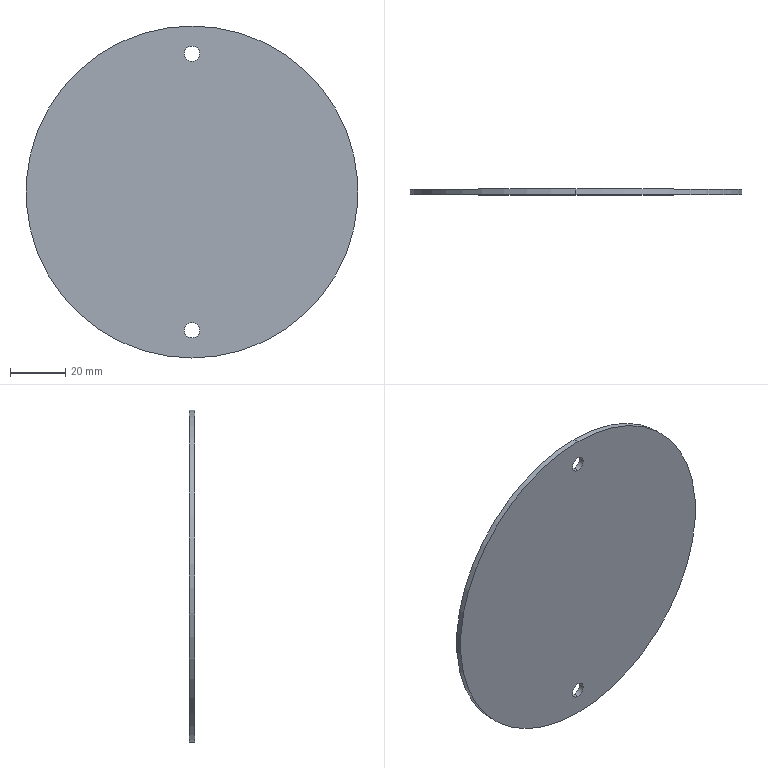Component | SolidWorks | YC1-25-01-08OilHoleCover-1 | 1 solid | 8 faces | box 120 x 2 x 120 mm | volume 22524 mm3 | cylinder 6 | plane 2 | commonest cylinder face diameters 5.5 x4 120 x2 | material Plain Carbon Steel
STEP:
#1=CARTESIAN_POINT('',(-19.291,153.78,-19.665));
#2=VERTEX_POINT('',#1);
#3=CARTESIAN_POINT('',(-19.291,153.78,-24.39));
#4=VERTEX_POINT('',#3);
#5=CARTESIAN_POINT('',(-19.291,153.78,-22.028));
#6=DIRECTION('',(0.,1.,0.));
#7=DIRECTION('',(0.,0.,-1.));
#8=AXIS2_PLACEMENT_3D('',#5,#6,#7);
#9=CIRCLE('',#8,2.362);
#10=EDGE_CURVE('',#2,#4,#9,.T.);
#11=ORIENTED_EDGE('',*,*,#10,.F.);
#12=CARTESIAN_POINT('',(-19.291,153.701,-19.665));
#13=VERTEX_POINT('',#12);
#14=CARTESIAN_POINT('',(-19.291,153.78,-19.665));
#15=DIRECTION('',(0.,-1.,0.));
#16=VECTOR('',#15,39.37);
#17=LINE('',#14,#16);
#18=EDGE_CURVE('',#2,#13,#17,.T.);
#19=ORIENTED_EDGE('',*,*,#18,.T.);
#20=CARTESIAN_POINT('',(-19.291,153.701,-24.39));
#21=VERTEX_POINT('',#20);
#22=CARTESIAN_POINT('',(-19.291,153.701,-22.028));
#23=DIRECTION('',(0.,1.,0.));
#24=DIRECTION('',(0.,0.,-1.));
#25=AXIS2_PLACEMENT_3D('',#22,#23,#24);
#26=CIRCLE('',#25,2.362);
#27=EDGE_CURVE('',#13,#21,#26,.T.);
#28=ORIENTED_EDGE('',*,*,#27,.T.);
#29=CARTESIAN_POINT('',(-19.291,153.78,-24.39));
#30=DIRECTION('',(0.,-1.,0.));
#31=VECTOR('',#30,39.37);
#32=LINE('',#29,#31);
#33=EDGE_CURVE('',#4,#21,#32,.T.);
#34=ORIENTED_EDGE('',*,*,#33,.F.);
#35=EDGE_LOOP('',(#11,#19,#28,#34));
#36=FACE_OUTER_BOUND('',#35,.T.);
#37=CARTESIAN_POINT('',(-19.291,153.78,-22.028));
#38=DIRECTION('',(0.,-1.,0.));
#39=DIRECTION('',(0.,0.,-1.));
#40=AXIS2_PLACEMENT_3D('',#37,#38,#39);
#41=CYLINDRICAL_SURFACE('',#40,2.362);
#42=ADVANCED_FACE('',(#36),#41,.T.);
#43=CARTESIAN_POINT('',(-19.291,153.701,-24.104));
#44=VERTEX_POINT('',#43);
#45=CARTESIAN_POINT('',(-19.291,153.701,-23.888));
#46=VERTEX_POINT('',#45);
#47=CARTESIAN_POINT('',(-19.291,153.701,-23.996));
#48=DIRECTION('',(0.,1.,0.));
#49=DIRECTION('',(0.,0.,1.));
#50=AXIS2_PLACEMENT_3D('',#47,#48,#49);
#51=CIRCLE('',#50,0.1083);
#52=EDGE_CURVE('',#44,#46,#51,.T.);
#53=ORIENTED_EDGE('',*,*,#52,.F.);
#54=CARTESIAN_POINT('',(-19.291,153.78,-24.104));
#55=VERTEX_POINT('',#54);
#56=CARTESIAN_POINT('',(-19.291,153.78,-24.104));
#57=DIRECTION('',(0.,1.,0.));
#58=VECTOR('',#57,39.37);
#59=LINE('',#56,#58);
#60=EDGE_CURVE('',#44,#55,#59,.T.);
#61=ORIENTED_EDGE('',*,*,#60,.T.);
#62=CARTESIAN_POINT('',(-19.291,153.78,-23.888));
#63=VERTEX_POINT('',#62);
#64=CARTESIAN_POINT('',(-19.291,153.78,-23.996));
#65=DIRECTION('',(0.,-1.,0.));
#66=DIRECTION('',(0.,0.,1.));
#67=AXIS2_PLACEMENT_3D('',#64,#65,#66);
#68=CIRCLE('',#67,0.1083);
#69=EDGE_CURVE('',#63,#55,#68,.T.);
#70=ORIENTED_EDGE('',*,*,#69,.F.);
#71=CARTESIAN_POINT('',(-19.291,153.78,-23.888));
#72=DIRECTION('',(0.,1.,0.));
#73=VECTOR('',#72,39.37);
#74=LINE('',#71,#73);
#75=EDGE_CURVE('',#46,#63,#74,.T.);
#76=ORIENTED_EDGE('',*,*,#75,.F.);
#77=EDGE_LOOP('',(#53,#61,#70,#76));
#78=FACE_OUTER_BOUND('',#77,.T.);
#79=CARTESIAN_POINT('',(-19.291,153.78,-23.996));
#80=DIRECTION('',(0.,1.,0.));
#81=DIRECTION('',(0.,0.,1.));
#82=AXIS2_PLACEMENT_3D('',#79,#80,#81);
#83=CYLINDRICAL_SURFACE('',#82,0.1083);
#84=ADVANCED_FACE('',(#78),#83,.F.);
#85=CARTESIAN_POINT('',(-19.291,153.701,-20.167));
#86=VERTEX_POINT('',#85);
#87=CARTESIAN_POINT('',(-19.291,153.701,-19.951));
#88=VERTEX_POINT('',#87);
#89=CARTESIAN_POINT('',(-19.291,153.701,-20.059));
#90=DIRECTION('',(0.,1.,0.));
#91=DIRECTION('',(0.,0.,1.));
#92=AXIS2_PLACEMENT_3D('',#89,#90,#91);
#93=CIRCLE('',#92,0.1083);
#94=EDGE_CURVE('',#86,#88,#93,.T.);
#95=ORIENTED_EDGE('',*,*,#94,.F.);
#96=CARTESIAN_POINT('',(-19.291,153.78,-20.167));
#97=VERTEX_POINT('',#96);
#98=CARTESIAN_POINT('',(-19.291,153.78,-20.167));
#99=DIRECTION('',(0.,1.,0.));
#100=VECTOR('',#99,39.37);
#101=LINE('',#98,#100);
#102=EDGE_CURVE('',#86,#97,#101,.T.);
#103=ORIENTED_EDGE('',*,*,#102,.T.);
#104=CARTESIAN_POINT('',(-19.291,153.78,-19.951));
#105=VERTEX_POINT('',#104);
#106=CARTESIAN_POINT('',(-19.291,153.78,-20.059));
#107=DIRECTION('',(0.,-1.,0.));
#108=DIRECTION('',(0.,0.,1.));
#109=AXIS2_PLACEMENT_3D('',#106,#107,#108);
#110=CIRCLE('',#109,0.1083);
#111=EDGE_CURVE('',#105,#97,#110,.T.);
#112=ORIENTED_EDGE('',*,*,#111,.F.);
#113=CARTESIAN_POINT('',(-19.291,153.78,-19.951));
#114=DIRECTION('',(0.,1.,0.));
#115=VECTOR('',#114,39.37);
#116=LINE('',#113,#115);
#117=EDGE_CURVE('',#88,#105,#116,.T.);
#118=ORIENTED_EDGE('',*,*,#117,.F.);
#119=EDGE_LOOP('',(#95,#103,#112,#118));
#120=FACE_OUTER_BOUND('',#119,.T.);
#121=CARTESIAN_POINT('',(-19.291,153.78,-20.059));
#122=DIRECTION('',(0.,1.,0.));
#123=DIRECTION('',(0.,0.,1.));
#124=AXIS2_PLACEMENT_3D('',#121,#122,#123);
#125=CYLINDRICAL_SURFACE('',#124,0.1083);
#126=ADVANCED_FACE('',(#120),#125,.F.);
#127=CARTESIAN_POINT('',(-19.291,153.78,-22.028));
#128=DIRECTION('',(0.,1.,0.));
#129=DIRECTION('',(0.,0.,-1.));
#130=AXIS2_PLACEMENT_3D('',#127,#128,#129);
#131=CIRCLE('',#130,2.362);
#132=EDGE_CURVE('',#4,#2,#131,.T.);
#133=ORIENTED_EDGE('',*,*,#132,.T.);
#134=ORIENTED_EDGE('',*,*,#10,.T.);
#135=EDGE_LOOP('',(#133,#134));
#136=FACE_OUTER_BOUND('',#135,.T.);
#137=ORIENTED_EDGE('',*,*,#69,.T.);
#138=CARTESIAN_POINT('',(-19.291,153.78,-23.996));
#139=DIRECTION('',(0.,-1.,0.));
#140=DIRECTION('',(0.,0.,1.));
#141=AXIS2_PLACEMENT_3D('',#138,#139,#140);
#142=CIRCLE('',#141,0.1083);
#143=EDGE_CURVE('',#55,#63,#142,.T.);
#144=ORIENTED_EDGE('',*,*,#143,.T.);
#145=EDGE_LOOP('',(#137,#144));
#146=FACE_BOUND('',#145,.T.);
#147=ORIENTED_EDGE('',*,*,#111,.T.);
#148=CARTESIAN_POINT('',(-19.291,153.78,-20.059));
#149=DIRECTION('',(0.,-1.,0.));
#150=DIRECTION('',(0.,0.,1.));
#151=AXIS2_PLACEMENT_3D('',#148,#149,#150);
#152=CIRCLE('',#151,0.1083);
#153=EDGE_CURVE('',#97,#105,#152,.T.);
#154=ORIENTED_EDGE('',*,*,#153,.T.);
#155=EDGE_LOOP('',(#147,#154));
#156=FACE_BOUND('',#155,.T.);
#157=CARTESIAN_POINT('',(-19.291,153.78,-22.028));
#158=DIRECTION('',(0.,1.,0.));
#159=DIRECTION('',(0.,0.,1.));
#160=AXIS2_PLACEMENT_3D('',#157,#158,#159);
#161=PLANE('',#160);
#162=ADVANCED_FACE('',(#136,#146,#156),#161,.T.);
#163=ORIENTED_EDGE('',*,*,#18,.F.);
#164=ORIENTED_EDGE('',*,*,#132,.F.);
#165=ORIENTED_EDGE('',*,*,#33,.T.);
#166=CARTESIAN_POINT('',(-19.291,153.701,-22.028));
#167=DIRECTION('',(0.,1.,0.));
#168=DIRECTION('',(0.,0.,-1.));
#169=AXIS2_PLACEMENT_3D('',#166,#167,#168);
#170=CIRCLE('',#169,2.362);
#171=EDGE_CURVE('',#21,#13,#170,.T.);
#172=ORIENTED_EDGE('',*,*,#171,.T.);
#173=EDGE_LOOP('',(#163,#164,#165,#172));
#174=FACE_OUTER_BOUND('',#173,.T.);
#175=CARTESIAN_POINT('',(-19.291,153.78,-22.028));
#176=DIRECTION('',(0.,-1.,0.));
#177=DIRECTION('',(0.,0.,-1.));
#178=AXIS2_PLACEMENT_3D('',#175,#176,#177);
#179=CYLINDRICAL_SURFACE('',#178,2.362);
#180=ADVANCED_FACE('',(#174),#179,.T.);
#181=ORIENTED_EDGE('',*,*,#60,.F.);
#182=CARTESIAN_POINT('',(-19.291,153.701,-23.996));
#183=DIRECTION('',(0.,1.,0.));
#184=DIRECTION('',(0.,0.,1.));
#185=AXIS2_PLACEMENT_3D('',#182,#183,#184);
#186=CIRCLE('',#185,0.1083);
#187=EDGE_CURVE('',#46,#44,#186,.T.);
#188=ORIENTED_EDGE('',*,*,#187,.F.);
#189=ORIENTED_EDGE('',*,*,#75,.T.);
#190=ORIENTED_EDGE('',*,*,#143,.F.);
#191=EDGE_LOOP('',(#181,#188,#189,#190));
#192=FACE_OUTER_BOUND('',#191,.T.);
#193=CARTESIAN_POINT('',(-19.291,153.78,-23.996));
#194=DIRECTION('',(0.,1.,0.));
#195=DIRECTION('',(0.,0.,1.));
#196=AXIS2_PLACEMENT_3D('',#193,#194,#195);
#197=CYLINDRICAL_SURFACE('',#196,0.1083);
#198=ADVANCED_FACE('',(#192),#197,.F.);
#199=ORIENTED_EDGE('',*,*,#102,.F.);
#200=CARTESIAN_POINT('',(-19.291,153.701,-20.059));
#201=DIRECTION('',(0.,1.,0.));
#202=DIRECTION('',(0.,0.,1.));
#203=AXIS2_PLACEMENT_3D('',#200,#201,#202);
#204=CIRCLE('',#203,0.1083);
#205=EDGE_CURVE('',#88,#86,#204,.T.);
#206=ORIENTED_EDGE('',*,*,#205,.F.);
#207=ORIENTED_EDGE('',*,*,#117,.T.);
#208=ORIENTED_EDGE('',*,*,#153,.F.);
#209=EDGE_LOOP('',(#199,#206,#207,#208));
#210=FACE_OUTER_BOUND('',#209,.T.);
#211=CARTESIAN_POINT('',(-19.291,153.78,-20.059));
#212=DIRECTION('',(0.,1.,0.));
#213=DIRECTION('',(0.,0.,1.));
#214=AXIS2_PLACEMENT_3D('',#211,#212,#213);
#215=CYLINDRICAL_SURFACE('',#214,0.1083);
#216=ADVANCED_FACE('',(#210),#215,.F.);
#217=ORIENTED_EDGE('',*,*,#171,.F.);
#218=ORIENTED_EDGE('',*,*,#27,.F.);
#219=EDGE_LOOP('',(#217,#218));
#220=FACE_OUTER_BOUND('',#219,.T.);
#221=ORIENTED_EDGE('',*,*,#187,.T.);
#222=ORIENTED_EDGE('',*,*,#52,.T.);
#223=EDGE_LOOP('',(#221,#222));
#224=FACE_BOUND('',#223,.T.);
#225=ORIENTED_EDGE('',*,*,#205,.T.);
#226=ORIENTED_EDGE('',*,*,#94,.T.);
#227=EDGE_LOOP('',(#225,#226));
#228=FACE_BOUND('',#227,.T.);
#229=CARTESIAN_POINT('',(-19.291,153.701,-22.028));
#230=DIRECTION('',(0.,1.,0.));
#231=DIRECTION('',(0.,0.,1.));
#232=AXIS2_PLACEMENT_3D('',#229,#230,#231);
#233=PLANE('',#232);
#234=ADVANCED_FACE('',(#220,#224,#228),#233,.F.);
#235=CLOSED_SHELL('',(#42,#84,#126,#162,#180,#198,#216,#234));
#236=MANIFOLD_SOLID_BREP('',#235);
#237=CARTESIAN_POINT('',(0.,0.,0.));
#238=DIRECTION('',(0.,0.,1.));
#239=DIRECTION('',(1.,0.,0.));
#240=AXIS2_PLACEMENT_3D('',#237,#238,#239);
#241=(LENGTH_UNIT()NAMED_UNIT(*)SI_UNIT($,.METRE.));
#242=LENGTH_MEASURE_WITH_UNIT(LENGTH_MEASURE(0.0254),#241);
#243=DIMENSIONAL_EXPONENTS(1.,0.,0.,0.,0.,0.,0.);
#244=(CONVERSION_BASED_UNIT('',#242)LENGTH_UNIT()NAMED_UNIT(#243));
#245=UNCERTAINTY_MEASURE_WITH_UNIT(LENGTH_MEASURE(0.00001),#244,'','');
#246=(NAMED_UNIT(*)PLANE_ANGLE_UNIT()SI_UNIT($,.RADIAN.));
#247=(NAMED_UNIT(*)SI_UNIT($,.STERADIAN.)SOLID_ANGLE_UNIT());
#248=(GEOMETRIC_REPRESENTATION_CONTEXT(3)GLOBAL_UNCERTAINTY_ASSIGNED_CONTEXT((#245))GLOBAL_UNIT_ASSIGNED_CONTEXT((#244,#246,#247))REPRESENTATION_CONTEXT('',''));
#249=ADVANCED_BREP_SHAPE_REPRESENTATION('',(#236,#240),#248);
#250=COLOUR_RGB('',0.7922,0.8196,0.9333);
#251=FILL_AREA_STYLE_COLOUR('',#250);
#252=FILL_AREA_STYLE('',(#251));
#253=SURFACE_STYLE_FILL_AREA(#252);
#254=SURFACE_SIDE_STYLE('',(#253));
#255=SURFACE_STYLE_USAGE(.BOTH.,#254);
#256=PRESENTATION_STYLE_ASSIGNMENT((#255));
#257=STYLED_ITEM('',(#256),#236);
#258=PRESENTATION_LAYER_ASSIGNMENT('','',(#257));
#259=(LENGTH_UNIT()NAMED_UNIT(*)SI_UNIT($,.METRE.));
#260=LENGTH_MEASURE_WITH_UNIT(LENGTH_MEASURE(0.0254),#259);
#261=DIMENSIONAL_EXPONENTS(1.,0.,0.,0.,0.,0.,0.);
#262=(CONVERSION_BASED_UNIT('',#260)LENGTH_UNIT()NAMED_UNIT(#261));
#263=UNCERTAINTY_MEASURE_WITH_UNIT(LENGTH_MEASURE(0.00001),#262,'','');
#264=(NAMED_UNIT(*)PLANE_ANGLE_UNIT()SI_UNIT($,.RADIAN.));
#265=(NAMED_UNIT(*)SI_UNIT($,.STERADIAN.)SOLID_ANGLE_UNIT());
#266=(GEOMETRIC_REPRESENTATION_CONTEXT(3)GLOBAL_UNCERTAINTY_ASSIGNED_CONTEXT((#263))GLOBAL_UNIT_ASSIGNED_CONTEXT((#262,#264,#265))REPRESENTATION_CONTEXT('',''));
#267=MECHANICAL_DESIGN_GEOMETRIC_PRESENTATION_REPRESENTATION('',(#257),#266);